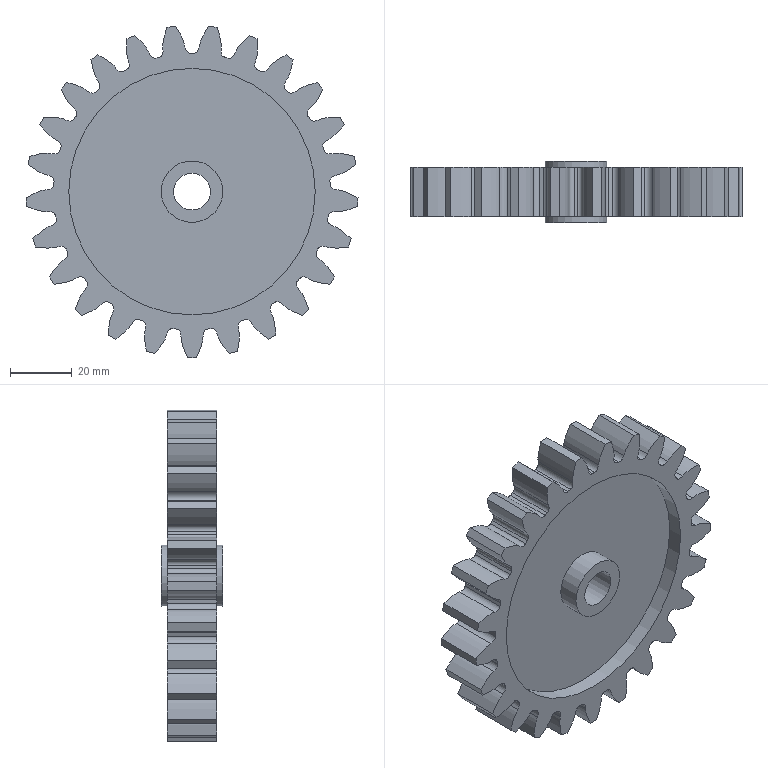Component | NX | GUIDE_GEAR | 1 solid | 161 faces | volume 75132 mm3 | spline 125 | cylinder 30 | plane 6 | commonest cylinder face diameters 89.84 x25 80 x2 20 x2 12 x1